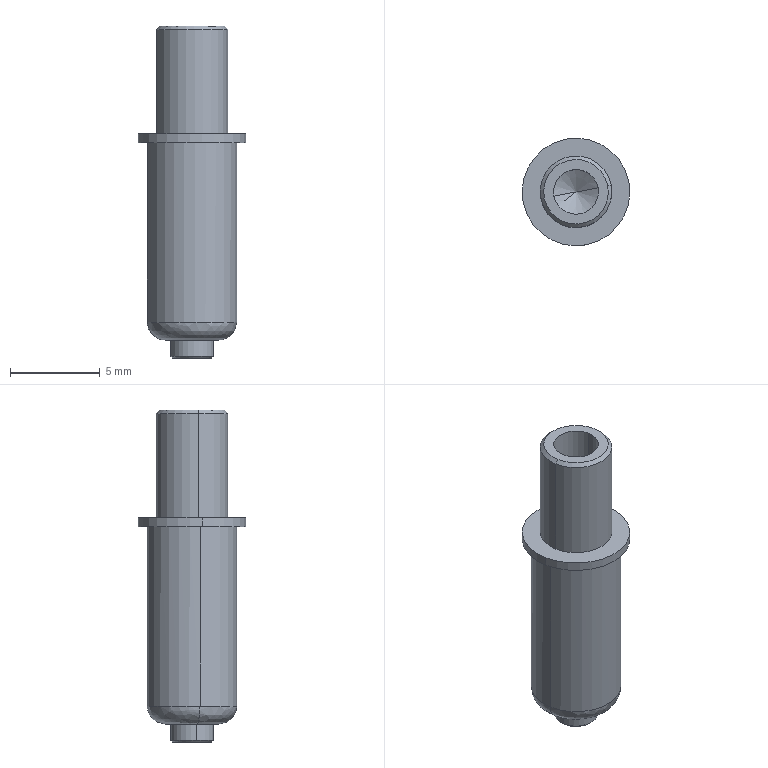Component | SolidWorks | F01AE00111-A2000-21TopEdgeAssembly-1_F01AE00111-A2000-19TopEdgeRollerAssembly-1_ElasticPIN5N--1 | 1 solid | 23 faces | box 6 x 6 x 18.5 mm | volume 274 mm3 | cylinder 10 | cone 6 | plane 5 | spline 2 | commonest cylinder face diameters 2.5 x2 4 x2 5 x2 6 x2 2.4 x2
STEP:
#1=CARTESIAN_POINT('',(-5.052,3.469,-15.668));
#2=VERTEX_POINT('',#1);
#3=CARTESIAN_POINT('',(-4.936,3.491,-15.668));
#4=VERTEX_POINT('',#3);
#5=CARTESIAN_POINT('',(-5.052,3.469,-15.668));
#6=CARTESIAN_POINT('',(-5.03,3.355,-15.668));
#7=CARTESIAN_POINT('',(-4.916,3.376,-15.668));
#8=CARTESIAN_POINT('',(-4.936,3.491,-15.668));
#9=(BOUNDED_CURVE()B_SPLINE_CURVE(3,(#5,#6,#7,#8),.UNSPECIFIED.,.F.,.T.)B_SPLINE_CURVE_WITH_KNOTS((4,4),(0.,0.9952),.UNSPECIFIED.)CURVE()GEOMETRIC_REPRESENTATION_ITEM()RATIONAL_B_SPLINE_CURVE((1.,0.3384,0.3384,1.))REPRESENTATION_ITEM(''));
#10=EDGE_CURVE('',#2,#4,#9,.T.);
#11=ORIENTED_EDGE('',*,*,#10,.T.);
#12=CARTESIAN_POINT('',(-4.897,3.498,-15.629));
#13=VERTEX_POINT('',#12);
#14=CARTESIAN_POINT('',(-4.936,3.491,-15.629));
#15=DIRECTION('',(0.1761,-0.9844,-0.));
#16=DIRECTION('',(0.9844,0.1761,0.));
#17=AXIS2_PLACEMENT_3D('',#14,#15,#16);
#18=CIRCLE('',#17,0.03937);
#19=EDGE_CURVE('',#4,#13,#18,.T.);
#20=ORIENTED_EDGE('',*,*,#19,.T.);
#21=CARTESIAN_POINT('',(-5.091,3.462,-15.629));
#22=VERTEX_POINT('',#21);
#23=CARTESIAN_POINT('',(-4.994,3.481,-15.629));
#24=DIRECTION('',(-0.,-0.,1.));
#25=DIRECTION('',(-0.9816,-0.1909,0.));
#26=AXIS2_PLACEMENT_3D('',#23,#24,#25);
#27=CIRCLE('',#26,0.09843);
#28=EDGE_CURVE('',#22,#13,#27,.T.);
#29=ORIENTED_EDGE('',*,*,#28,.F.);
#30=CARTESIAN_POINT('',(-5.091,3.463,-15.629));
#31=VERTEX_POINT('',#30);
#32=CARTESIAN_POINT('',(-4.994,3.481,-15.629));
#33=DIRECTION('',(-0.,-0.,1.));
#34=DIRECTION('',(-0.9816,-0.1909,0.));
#35=AXIS2_PLACEMENT_3D('',#32,#33,#34);
#36=CIRCLE('',#35,0.09843);
#37=EDGE_CURVE('',#31,#22,#36,.T.);
#38=ORIENTED_EDGE('',*,*,#37,.F.);
#39=CARTESIAN_POINT('',(-5.052,3.47,-15.668));
#40=VERTEX_POINT('',#39);
#41=CARTESIAN_POINT('',(-5.052,3.47,-15.629));
#42=DIRECTION('',(-0.1761,0.9844,0.));
#43=DIRECTION('',(-0.9844,-0.1761,0.));
#44=AXIS2_PLACEMENT_3D('',#41,#42,#43);
#45=CIRCLE('',#44,0.03937);
#46=EDGE_CURVE('',#40,#31,#45,.T.);
#47=ORIENTED_EDGE('',*,*,#46,.F.);
#48=CARTESIAN_POINT('',(-5.052,3.469,-15.668));
#49=CARTESIAN_POINT('',(-5.052,3.47,-15.668));
#50=CARTESIAN_POINT('',(-5.052,3.47,-15.668));
#51=CARTESIAN_POINT('',(-5.052,3.47,-15.668));
#52=B_SPLINE_CURVE_WITH_KNOTS('',3,(#48,#49,#50,#51),.UNSPECIFIED.,.F.,.F.,(4,4),(0.,0.004937),.UNSPECIFIED.);
#53=EDGE_CURVE('',#2,#40,#52,.T.);
#54=ORIENTED_EDGE('',*,*,#53,.F.);
#55=EDGE_LOOP('',(#11,#20,#29,#38,#47,#54));
#56=FACE_OUTER_BOUND('',#55,.T.);
#57=CARTESIAN_POINT('',(-4.936,3.491,-15.668));
#58=CARTESIAN_POINT('',(-4.93,3.457,-15.668));
#59=CARTESIAN_POINT('',(-4.95,3.429,-15.668));
#60=CARTESIAN_POINT('',(-4.984,3.423,-15.668));
#61=CARTESIAN_POINT('',(-5.018,3.417,-15.668));
#62=CARTESIAN_POINT('',(-5.046,3.436,-15.668));
#63=CARTESIAN_POINT('',(-5.052,3.47,-15.668));
#64=CARTESIAN_POINT('',(-4.914,3.495,-15.669));
#65=CARTESIAN_POINT('',(-4.905,3.448,-15.669));
#66=CARTESIAN_POINT('',(-4.933,3.408,-15.669));
#67=CARTESIAN_POINT('',(-4.98,3.4,-15.669));
#68=CARTESIAN_POINT('',(-5.027,3.392,-15.669));
#69=CARTESIAN_POINT('',(-5.066,3.419,-15.669));
#70=CARTESIAN_POINT('',(-5.075,3.466,-15.669));
#71=CARTESIAN_POINT('',(-4.897,3.498,-15.652));
#72=CARTESIAN_POINT('',(-4.887,3.441,-15.652));
#73=CARTESIAN_POINT('',(-4.92,3.394,-15.652));
#74=CARTESIAN_POINT('',(-4.977,3.384,-15.652));
#75=CARTESIAN_POINT('',(-5.034,3.374,-15.652));
#76=CARTESIAN_POINT('',(-5.081,3.407,-15.652));
#77=CARTESIAN_POINT('',(-5.091,3.463,-15.652));
#78=CARTESIAN_POINT('',(-4.897,3.498,-15.629));
#79=CARTESIAN_POINT('',(-4.887,3.441,-15.629));
#80=CARTESIAN_POINT('',(-4.92,3.394,-15.629));
#81=CARTESIAN_POINT('',(-4.977,3.384,-15.629));
#82=CARTESIAN_POINT('',(-5.034,3.374,-15.629));
#83=CARTESIAN_POINT('',(-5.081,3.407,-15.629));
#84=CARTESIAN_POINT('',(-5.091,3.463,-15.629));
#85=(BOUNDED_SURFACE()B_SPLINE_SURFACE(3,3,((#57,#58,#59,#60,#61,#62,#63),(#64,#65,#66,#67,#68,#69,#70),(#71,#72,#73,#74,#75,#76,#77),(#78,#79,#80,#81,#82,#83,#84)),.UNSPECIFIED.,.F.,.F.,.T.)B_SPLINE_SURFACE_WITH_KNOTS((4,4),(4,3,4),(0.,1.),(0.,0.5,1.),.UNSPECIFIED.)GEOMETRIC_REPRESENTATION_ITEM()RATIONAL_B_SPLINE_SURFACE(((1.,0.8047,0.8047,1.,0.8047,0.8047,1.),(0.8025,0.6458,0.6458,0.8025,0.6458,0.6458,0.8025),(0.8025,0.6458,0.6458,0.8025,0.6458,0.6458,0.8025),(1.,0.8047,0.8047,1.,0.8047,0.8047,1.)))REPRESENTATION_ITEM('')SURFACE());
#86=ADVANCED_FACE('',(#56),#85,.T.);
#87=CARTESIAN_POINT('',(-4.925,3.494,-14.979));
#88=VERTEX_POINT('',#87);
#89=CARTESIAN_POINT('',(-5.064,3.467,-14.979));
#90=VERTEX_POINT('',#89);
#91=CARTESIAN_POINT('',(-4.994,3.481,-14.979));
#92=DIRECTION('',(-0.,-0.,1.));
#93=DIRECTION('',(0.9816,0.1909,0.));
#94=AXIS2_PLACEMENT_3D('',#91,#92,#93);
#95=CIRCLE('',#94,0.07087);
#96=EDGE_CURVE('',#88,#90,#95,.T.);
#97=ORIENTED_EDGE('',*,*,#96,.F.);
#98=CARTESIAN_POINT('',(-4.917,3.496,-14.987));
#99=VERTEX_POINT('',#98);
#100=CARTESIAN_POINT('',(-4.925,3.494,-14.979));
#101=DIRECTION('',(0.6941,0.135,-0.7071));
#102=VECTOR('',#101,39.37);
#103=LINE('',#100,#102);
#104=EDGE_CURVE('',#88,#99,#103,.T.);
#105=ORIENTED_EDGE('',*,*,#104,.T.);
#106=CARTESIAN_POINT('',(-5.071,3.466,-14.987));
#107=VERTEX_POINT('',#106);
#108=CARTESIAN_POINT('',(-4.994,3.481,-14.987));
#109=DIRECTION('',(0.,0.,-1.));
#110=DIRECTION('',(0.9816,0.1909,0.));
#111=AXIS2_PLACEMENT_3D('',#108,#109,#110);
#112=CIRCLE('',#111,0.07874);
#113=EDGE_CURVE('',#107,#99,#112,.T.);
#114=ORIENTED_EDGE('',*,*,#113,.F.);
#115=CARTESIAN_POINT('',(-5.064,3.467,-14.979));
#116=DIRECTION('',(-0.6941,-0.135,-0.7071));
#117=VECTOR('',#116,39.37);
#118=LINE('',#115,#117);
#119=EDGE_CURVE('',#90,#107,#118,.T.);
#120=ORIENTED_EDGE('',*,*,#119,.F.);
#121=EDGE_LOOP('',(#97,#105,#114,#120));
#122=FACE_OUTER_BOUND('',#121,.T.);
#123=CARTESIAN_POINT('',(-4.994,3.481,-14.979));
#124=DIRECTION('',(0.,0.,-1.));
#125=DIRECTION('',(-0.9816,-0.1909,0.));
#126=AXIS2_PLACEMENT_3D('',#123,#124,#125);
#127=CONICAL_SURFACE('',#126,0.07087,0.7854);
#128=ADVANCED_FACE('',(#122),#127,.T.);
#129=CARTESIAN_POINT('',(-5.042,3.471,-15.235));
#130=VERTEX_POINT('',#129);
#131=CARTESIAN_POINT('',(-4.946,3.49,-15.235));
#132=VERTEX_POINT('',#131);
#133=CARTESIAN_POINT('',(-4.994,3.481,-15.235));
#134=DIRECTION('',(-0.,-0.,1.));
#135=DIRECTION('',(0.9816,0.1909,0.));
#136=AXIS2_PLACEMENT_3D('',#133,#134,#135);
#137=CIRCLE('',#136,0.04921);
#138=EDGE_CURVE('',#130,#132,#137,.T.);
#139=ORIENTED_EDGE('',*,*,#138,.F.);
#140=CARTESIAN_POINT('',(-5.042,3.471,-14.979));
#141=VERTEX_POINT('',#140);
#142=CARTESIAN_POINT('',(-5.042,3.471,-14.979));
#143=DIRECTION('',(-0.,-0.,1.));
#144=VECTOR('',#143,39.37);
#145=LINE('',#142,#144);
#146=EDGE_CURVE('',#130,#141,#145,.T.);
#147=ORIENTED_EDGE('',*,*,#146,.T.);
#148=CARTESIAN_POINT('',(-4.946,3.49,-14.979));
#149=VERTEX_POINT('',#148);
#150=CARTESIAN_POINT('',(-4.994,3.481,-14.979));
#151=DIRECTION('',(-0.,-0.,1.));
#152=DIRECTION('',(0.9816,0.1909,0.));
#153=AXIS2_PLACEMENT_3D('',#150,#151,#152);
#154=CIRCLE('',#153,0.04921);
#155=EDGE_CURVE('',#141,#149,#154,.T.);
#156=ORIENTED_EDGE('',*,*,#155,.T.);
#157=CARTESIAN_POINT('',(-4.946,3.49,-14.979));
#158=DIRECTION('',(-0.,-0.,1.));
#159=VECTOR('',#158,39.37);
#160=LINE('',#157,#159);
#161=EDGE_CURVE('',#132,#149,#160,.T.);
#162=ORIENTED_EDGE('',*,*,#161,.F.);
#163=EDGE_LOOP('',(#139,#147,#156,#162));
#164=FACE_OUTER_BOUND('',#163,.T.);
#165=CARTESIAN_POINT('',(-4.994,3.481,-14.979));
#166=DIRECTION('',(-0.,-0.,1.));
#167=DIRECTION('',(0.9816,0.1909,0.));
#168=AXIS2_PLACEMENT_3D('',#165,#166,#167);
#169=CYLINDRICAL_SURFACE('',#168,0.04921);
#170=ADVANCED_FACE('',(#164),#169,.F.);
#171=CARTESIAN_POINT('',(-4.994,3.481,-15.265));
#172=VERTEX_POINT('',#171);
#173=CARTESIAN_POINT('',(-4.946,3.49,-15.235));
#174=DIRECTION('',(0.8414,0.1637,0.515));
#175=VECTOR('',#174,39.37);
#176=LINE('',#173,#175);
#177=EDGE_CURVE('',#172,#132,#176,.T.);
#178=ORIENTED_EDGE('',*,*,#177,.F.);
#179=CARTESIAN_POINT('',(-5.042,3.471,-15.235));
#180=DIRECTION('',(-0.8414,-0.1637,0.515));
#181=VECTOR('',#180,39.37);
#182=LINE('',#179,#181);
#183=EDGE_CURVE('',#172,#130,#182,.T.);
#184=ORIENTED_EDGE('',*,*,#183,.T.);
#185=ORIENTED_EDGE('',*,*,#138,.T.);
#186=EDGE_LOOP('',(#178,#184,#185));
#187=FACE_OUTER_BOUND('',#186,.T.);
#188=CARTESIAN_POINT('',(-4.994,3.481,-15.235));
#189=DIRECTION('',(-0.,-0.,1.));
#190=DIRECTION('',(0.9816,0.1909,0.));
#191=AXIS2_PLACEMENT_3D('',#188,#189,#190);
#192=CONICAL_SURFACE('',#191,0.04921,1.03);
#193=ADVANCED_FACE('',(#187),#192,.F.);
#194=ORIENTED_EDGE('',*,*,#113,.T.);
#195=CARTESIAN_POINT('',(-4.917,3.496,-15.216));
#196=VERTEX_POINT('',#195);
#197=CARTESIAN_POINT('',(-4.917,3.496,-14.979));
#198=DIRECTION('',(0.,0.,-1.));
#199=VECTOR('',#198,39.37);
#200=LINE('',#197,#199);
#201=EDGE_CURVE('',#99,#196,#200,.T.);
#202=ORIENTED_EDGE('',*,*,#201,.T.);
#203=CARTESIAN_POINT('',(-5.071,3.466,-15.216));
#204=VERTEX_POINT('',#203);
#205=CARTESIAN_POINT('',(-4.994,3.481,-15.216));
#206=DIRECTION('',(-0.,-0.,1.));
#207=DIRECTION('',(-0.9816,-0.1909,0.));
#208=AXIS2_PLACEMENT_3D('',#205,#206,#207);
#209=CIRCLE('',#208,0.07874);
#210=EDGE_CURVE('',#196,#204,#209,.T.);
#211=ORIENTED_EDGE('',*,*,#210,.T.);
#212=CARTESIAN_POINT('',(-5.071,3.466,-14.979));
#213=DIRECTION('',(0.,0.,-1.));
#214=VECTOR('',#213,39.37);
#215=LINE('',#212,#214);
#216=EDGE_CURVE('',#107,#204,#215,.T.);
#217=ORIENTED_EDGE('',*,*,#216,.F.);
#218=EDGE_LOOP('',(#194,#202,#211,#217));
#219=FACE_OUTER_BOUND('',#218,.T.);
#220=CARTESIAN_POINT('',(-4.994,3.481,-14.979));
#221=DIRECTION('',(0.,0.,-1.));
#222=DIRECTION('',(-0.9816,-0.1909,0.));
#223=AXIS2_PLACEMENT_3D('',#220,#221,#222);
#224=CYLINDRICAL_SURFACE('',#223,0.07874);
#225=ADVANCED_FACE('',(#219),#224,.T.);
#226=CARTESIAN_POINT('',(-5.091,3.462,-15.235));
#227=VERTEX_POINT('',#226);
#228=CARTESIAN_POINT('',(-4.898,3.499,-15.235));
#229=VERTEX_POINT('',#228);
#230=CARTESIAN_POINT('',(-4.994,3.481,-15.235));
#231=DIRECTION('',(0.,0.,-1.));
#232=DIRECTION('',(-0.9816,-0.1909,0.));
#233=AXIS2_PLACEMENT_3D('',#230,#231,#232);
#234=CIRCLE('',#233,0.09843);
#235=EDGE_CURVE('',#227,#229,#234,.T.);
#236=ORIENTED_EDGE('',*,*,#235,.T.);
#237=CARTESIAN_POINT('',(-4.898,3.499,-15.629));
#238=VERTEX_POINT('',#237);
#239=CARTESIAN_POINT('',(-4.898,3.499,-14.777));
#240=DIRECTION('',(0.,0.,-1.));
#241=VECTOR('',#240,39.37);
#242=LINE('',#239,#241);
#243=EDGE_CURVE('',#229,#238,#242,.T.);
#244=ORIENTED_EDGE('',*,*,#243,.T.);
#245=CARTESIAN_POINT('',(-4.994,3.481,-15.629));
#246=DIRECTION('',(-0.,-0.,1.));
#247=DIRECTION('',(-0.9816,-0.1909,0.));
#248=AXIS2_PLACEMENT_3D('',#245,#246,#247);
#249=CIRCLE('',#248,0.09843);
#250=EDGE_CURVE('',#238,#31,#249,.T.);
#251=ORIENTED_EDGE('',*,*,#250,.T.);
#252=ORIENTED_EDGE('',*,*,#37,.T.);
#253=CARTESIAN_POINT('',(-5.091,3.462,-14.777));
#254=DIRECTION('',(0.,0.,-1.));
#255=VECTOR('',#254,39.37);
#256=LINE('',#253,#255);
#257=EDGE_CURVE('',#227,#22,#256,.T.);
#258=ORIENTED_EDGE('',*,*,#257,.F.);
#259=EDGE_LOOP('',(#236,#244,#251,#252,#258));
#260=FACE_OUTER_BOUND('',#259,.T.);
#261=CARTESIAN_POINT('',(-4.994,3.481,-14.777));
#262=DIRECTION('',(0.,0.,-1.));
#263=DIRECTION('',(-0.9816,-0.1909,0.));
#264=AXIS2_PLACEMENT_3D('',#261,#262,#263);
#265=CYLINDRICAL_SURFACE('',#264,0.09843);
#266=ADVANCED_FACE('',(#260),#265,.T.);
#267=CARTESIAN_POINT('',(-5.11,3.458,-15.216));
#268=VERTEX_POINT('',#267);
#269=CARTESIAN_POINT('',(-4.878,3.503,-15.216));
#270=VERTEX_POINT('',#269);
#271=CARTESIAN_POINT('',(-4.994,3.481,-15.216));
#272=DIRECTION('',(0.,0.,-1.));
#273=DIRECTION('',(-0.9816,-0.1909,0.));
#274=AXIS2_PLACEMENT_3D('',#271,#272,#273);
#275=CIRCLE('',#274,0.1181);
#276=EDGE_CURVE('',#268,#270,#275,.T.);
#277=ORIENTED_EDGE('',*,*,#276,.T.);
#278=CARTESIAN_POINT('',(-4.878,3.503,-15.235));
#279=VERTEX_POINT('',#278);
#280=CARTESIAN_POINT('',(-4.878,3.503,-14.777));
#281=DIRECTION('',(0.,0.,-1.));
#282=VECTOR('',#281,39.37);
#283=LINE('',#280,#282);
#284=EDGE_CURVE('',#270,#279,#283,.T.);
#285=ORIENTED_EDGE('',*,*,#284,.T.);
#286=CARTESIAN_POINT('',(-5.11,3.458,-15.235));
#287=VERTEX_POINT('',#286);
#288=CARTESIAN_POINT('',(-4.994,3.481,-15.235));
#289=DIRECTION('',(0.,0.,-1.));
#290=DIRECTION('',(-0.9816,-0.1909,0.));
#291=AXIS2_PLACEMENT_3D('',#288,#289,#290);
#292=CIRCLE('',#291,0.1181);
#293=EDGE_CURVE('',#287,#279,#292,.T.);
#294=ORIENTED_EDGE('',*,*,#293,.F.);
#295=CARTESIAN_POINT('',(-5.11,3.458,-14.777));
#296=DIRECTION('',(0.,0.,-1.));
#297=VECTOR('',#296,39.37);
#298=LINE('',#295,#297);
#299=EDGE_CURVE('',#268,#287,#298,.T.);
#300=ORIENTED_EDGE('',*,*,#299,.F.);
#301=EDGE_LOOP('',(#277,#285,#294,#300));
#302=FACE_OUTER_BOUND('',#301,.T.);
#303=CARTESIAN_POINT('',(-4.994,3.481,-14.777));
#304=DIRECTION('',(0.,0.,-1.));
#305=DIRECTION('',(-0.9816,-0.1909,0.));
#306=AXIS2_PLACEMENT_3D('',#303,#304,#305);
#307=CYLINDRICAL_SURFACE('',#306,0.1181);
#308=ADVANCED_FACE('',(#302),#307,.T.);
#309=CARTESIAN_POINT('',(-4.948,3.49,-15.668));
#310=VERTEX_POINT('',#309);
#311=CARTESIAN_POINT('',(-5.041,3.472,-15.668));
#312=VERTEX_POINT('',#311);
#313=CARTESIAN_POINT('',(-4.994,3.481,-15.668));
#314=DIRECTION('',(-0.,-0.,1.));
#315=DIRECTION('',(-0.9816,-0.1909,0.));
#316=AXIS2_PLACEMENT_3D('',#313,#314,#315);
#317=CIRCLE('',#316,0.04724);
#318=EDGE_CURVE('',#310,#312,#317,.T.);
#319=ORIENTED_EDGE('',*,*,#318,.F.);
#320=CARTESIAN_POINT('',(-4.948,3.49,-15.704));
#321=VERTEX_POINT('',#320);
#322=CARTESIAN_POINT('',(-4.948,3.49,-14.777));
#323=DIRECTION('',(0.,0.,-1.));
#324=VECTOR('',#323,39.37);
#325=LINE('',#322,#324);
#326=EDGE_CURVE('',#310,#321,#325,.T.);
#327=ORIENTED_EDGE('',*,*,#326,.T.);
#328=CARTESIAN_POINT('',(-5.041,3.472,-15.704));
#329=VERTEX_POINT('',#328);
#330=CARTESIAN_POINT('',(-4.994,3.481,-15.704));
#331=DIRECTION('',(-0.,-0.,1.));
#332=DIRECTION('',(-0.9816,-0.1909,0.));
#333=AXIS2_PLACEMENT_3D('',#330,#331,#332);
#334=CIRCLE('',#333,0.04724);
#335=EDGE_CURVE('',#321,#329,#334,.T.);
#336=ORIENTED_EDGE('',*,*,#335,.T.);
#337=CARTESIAN_POINT('',(-5.041,3.472,-14.777));
#338=DIRECTION('',(0.,0.,-1.));
#339=VECTOR('',#338,39.37);
#340=LINE('',#337,#339);
#341=EDGE_CURVE('',#312,#329,#340,.T.);
#342=ORIENTED_EDGE('',*,*,#341,.F.);
#343=EDGE_LOOP('',(#319,#327,#336,#342));
#344=FACE_OUTER_BOUND('',#343,.T.);
#345=CARTESIAN_POINT('',(-4.994,3.481,-14.777));
#346=DIRECTION('',(0.,0.,-1.));
#347=DIRECTION('',(-0.9816,-0.1909,0.));
#348=AXIS2_PLACEMENT_3D('',#345,#346,#347);
#349=CYLINDRICAL_SURFACE('',#348,0.04724);
#350=ADVANCED_FACE('',(#344),#349,.T.);
#351=CARTESIAN_POINT('',(-4.952,3.489,-15.708));
#352=VERTEX_POINT('',#351);
#353=CARTESIAN_POINT('',(-5.037,3.472,-15.708));
#354=VERTEX_POINT('',#353);
#355=CARTESIAN_POINT('',(-4.994,3.481,-15.708));
#356=DIRECTION('',(-0.,-0.,1.));
#357=DIRECTION('',(0.9816,0.1909,0.));
#358=AXIS2_PLACEMENT_3D('',#355,#356,#357);
#359=CIRCLE('',#358,0.04331);
#360=EDGE_CURVE('',#352,#354,#359,.T.);
#361=ORIENTED_EDGE('',*,*,#360,.T.);
#362=CARTESIAN_POINT('',(-5.041,3.472,-15.704));
#363=DIRECTION('',(-0.6941,-0.135,0.7071));
#364=VECTOR('',#363,39.37);
#365=LINE('',#362,#364);
#366=EDGE_CURVE('',#354,#329,#365,.T.);
#367=ORIENTED_EDGE('',*,*,#366,.T.);
#368=ORIENTED_EDGE('',*,*,#335,.F.);
#369=CARTESIAN_POINT('',(-4.948,3.49,-15.704));
#370=DIRECTION('',(0.6941,0.135,0.7071));
#371=VECTOR('',#370,39.37);
#372=LINE('',#369,#371);
#373=EDGE_CURVE('',#352,#321,#372,.T.);
#374=ORIENTED_EDGE('',*,*,#373,.F.);
#375=EDGE_LOOP('',(#361,#367,#368,#374));
#376=FACE_OUTER_BOUND('',#375,.T.);
#377=CARTESIAN_POINT('',(-4.994,3.481,-15.704));
#378=DIRECTION('',(-0.,-0.,1.));
#379=DIRECTION('',(0.9816,0.1909,0.));
#380=AXIS2_PLACEMENT_3D('',#377,#378,#379);
#381=CONICAL_SURFACE('',#380,0.04724,0.7854);
#382=ADVANCED_FACE('',(#376),#381,.T.);
#383=ORIENTED_EDGE('',*,*,#276,.F.);
#384=CARTESIAN_POINT('',(-4.994,3.481,-15.216));
#385=DIRECTION('',(0.,0.,-1.));
#386=DIRECTION('',(-0.9816,-0.1909,0.));
#387=AXIS2_PLACEMENT_3D('',#384,#385,#386);
#388=CIRCLE('',#387,0.1181);
#389=EDGE_CURVE('',#270,#268,#388,.T.);
#390=ORIENTED_EDGE('',*,*,#389,.F.);
#391=EDGE_LOOP('',(#383,#390));
#392=FACE_OUTER_BOUND('',#391,.T.);
#393=CARTESIAN_POINT('',(-4.994,3.481,-15.216));
#394=DIRECTION('',(-0.,-0.,1.));
#395=DIRECTION('',(-0.9816,-0.1909,0.));
#396=AXIS2_PLACEMENT_3D('',#393,#394,#395);
#397=CIRCLE('',#396,0.07874);
#398=EDGE_CURVE('',#204,#196,#397,.T.);
#399=ORIENTED_EDGE('',*,*,#398,.F.);
#400=ORIENTED_EDGE('',*,*,#210,.F.);
#401=EDGE_LOOP('',(#399,#400));
#402=FACE_BOUND('',#401,.T.);
#403=CARTESIAN_POINT('',(-4.994,3.481,-15.216));
#404=DIRECTION('',(0.,0.,-1.));
#405=DIRECTION('',(-0.9816,-0.1909,-0.));
#406=AXIS2_PLACEMENT_3D('',#403,#404,#405);
#407=PLANE('',#406);
#408=ADVANCED_FACE('',(#392,#402),#407,.F.);
#409=ORIENTED_EDGE('',*,*,#243,.F.);
#410=CARTESIAN_POINT('',(-4.994,3.481,-15.235));
#411=DIRECTION('',(0.,0.,-1.));
#412=DIRECTION('',(-0.9816,-0.1909,0.));
#413=AXIS2_PLACEMENT_3D('',#410,#411,#412);
#414=CIRCLE('',#413,0.09843);
#415=EDGE_CURVE('',#229,#227,#414,.T.);
#416=ORIENTED_EDGE('',*,*,#415,.T.);
#417=ORIENTED_EDGE('',*,*,#257,.T.);
#418=ORIENTED_EDGE('',*,*,#28,.T.);
#419=CARTESIAN_POINT('',(-4.994,3.481,-15.629));
#420=DIRECTION('',(-0.,-0.,1.));
#421=DIRECTION('',(-0.9816,-0.1909,0.));
#422=AXIS2_PLACEMENT_3D('',#419,#420,#421);
#423=CIRCLE('',#422,0.09843);
#424=EDGE_CURVE('',#13,#238,#423,.T.);
#425=ORIENTED_EDGE('',*,*,#424,.T.);
#426=EDGE_LOOP('',(#409,#416,#417,#418,#425));
#427=FACE_OUTER_BOUND('',#426,.T.);
#428=CARTESIAN_POINT('',(-4.994,3.481,-14.777));
#429=DIRECTION('',(0.,0.,-1.));
#430=DIRECTION('',(-0.9816,-0.1909,0.));
#431=AXIS2_PLACEMENT_3D('',#428,#429,#430);
#432=CYLINDRICAL_SURFACE('',#431,0.09843);
#433=ADVANCED_FACE('',(#427),#432,.T.);
#434=ORIENTED_EDGE('',*,*,#19,.F.);
#435=CARTESIAN_POINT('',(-4.936,3.492,-15.668));
#436=VERTEX_POINT('',#435);
#437=CARTESIAN_POINT('',(-4.936,3.491,-15.668));
#438=CARTESIAN_POINT('',(-4.936,3.491,-15.668));
#439=CARTESIAN_POINT('',(-4.936,3.492,-15.668));
#440=CARTESIAN_POINT('',(-4.936,3.492,-15.668));
#441=(BOUNDED_CURVE()B_SPLINE_CURVE(3,(#437,#438,#439,#440),.UNSPECIFIED.,.F.,.T.)B_SPLINE_CURVE_WITH_KNOTS((4,4),(0.9952,1.),.UNSPECIFIED.)CURVE()GEOMETRIC_REPRESENTATION_ITEM()RATIONAL_B_SPLINE_CURVE((1.,1.,1.,1.))REPRESENTATION_ITEM(''));
#442=EDGE_CURVE('',#4,#436,#441,.T.);
#443=ORIENTED_EDGE('',*,*,#442,.T.);
#444=CARTESIAN_POINT('',(-5.052,3.47,-15.668));
#445=CARTESIAN_POINT('',(-5.053,3.474,-15.668));
#446=CARTESIAN_POINT('',(-5.053,3.479,-15.668));
#447=CARTESIAN_POINT('',(-5.053,3.485,-15.668));
#448=CARTESIAN_POINT('',(-5.053,3.489,-15.668));
#449=CARTESIAN_POINT('',(-5.052,3.49,-15.668));
#450=CARTESIAN_POINT('',(-5.05,3.5,-15.668));
#451=CARTESIAN_POINT('',(-5.047,3.508,-15.668));
#452=CARTESIAN_POINT('',(-5.04,3.518,-15.668));
#453=CARTESIAN_POINT('',(-5.037,3.522,-15.668));
#454=CARTESIAN_POINT('',(-5.031,3.527,-15.668));
#455=CARTESIAN_POINT('',(-5.029,3.528,-15.668));
#456=CARTESIAN_POINT('',(-5.027,3.53,-15.668));
#457=CARTESIAN_POINT('',(-5.026,3.53,-15.668));
#458=CARTESIAN_POINT('',(-5.019,3.535,-15.668));
#459=CARTESIAN_POINT('',(-5.012,3.537,-15.668));
#460=CARTESIAN_POINT('',(-5.001,3.539,-15.668));
#461=CARTESIAN_POINT('',(-4.996,3.54,-15.668));
#462=CARTESIAN_POINT('',(-4.989,3.54,-15.668));
#463=CARTESIAN_POINT('',(-4.987,3.539,-15.668));
#464=CARTESIAN_POINT('',(-4.985,3.539,-15.668));
#465=CARTESIAN_POINT('',(-4.984,3.539,-15.668));
#466=CARTESIAN_POINT('',(-4.975,3.537,-15.668));
#467=CARTESIAN_POINT('',(-4.968,3.534,-15.668));
#468=CARTESIAN_POINT('',(-4.958,3.527,-15.668));
#469=CARTESIAN_POINT('',(-4.953,3.523,-15.668));
#470=CARTESIAN_POINT('',(-4.948,3.518,-15.668));
#471=CARTESIAN_POINT('',(-4.947,3.516,-15.668));
#472=CARTESIAN_POINT('',(-4.945,3.514,-15.668));
#473=CARTESIAN_POINT('',(-4.945,3.513,-15.668));
#474=CARTESIAN_POINT('',(-4.94,3.506,-15.668));
#475=CARTESIAN_POINT('',(-4.938,3.499,-15.668));
#476=CARTESIAN_POINT('',(-4.936,3.492,-15.668));
#477=B_SPLINE_CURVE_WITH_KNOTS('',3,(#444,#445,#446,#447,#448,#449,#450,#451,#452,#453,#454,#455,#456,#457,#458,#459,#460,#461,#462,#463,#464,#465,#466,#467,#468,#469,#470,#471,#472,#473,#474,#475,#476),.UNSPECIFIED.,.F.,.F.,(4,1,2,2,2,1,1,2,2,2,1,1,2,2,2,1,1,2,2,4),(0.004937,0.06713,0.09822,0.1293,0.2537,0.3159,0.347,0.3625,0.3781,0.5025,0.5647,0.5958,0.6113,0.6269,0.7512,0.8134,0.8445,0.8601,0.8756,1.),.UNSPECIFIED.);
#478=EDGE_CURVE('',#40,#436,#477,.T.);
#479=ORIENTED_EDGE('',*,*,#478,.F.);
#480=ORIENTED_EDGE('',*,*,#46,.T.);
#481=ORIENTED_EDGE('',*,*,#250,.F.);
#482=ORIENTED_EDGE('',*,*,#424,.F.);
#483=EDGE_LOOP('',(#434,#443,#479,#480,#481,#482));
#484=FACE_OUTER_BOUND('',#483,.T.);
#485=CARTESIAN_POINT('',(-5.052,3.469,-15.668));
#486=CARTESIAN_POINT('',(-5.058,3.503,-15.668));
#487=CARTESIAN_POINT('',(-5.039,3.532,-15.668));
#488=CARTESIAN_POINT('',(-5.005,3.538,-15.668));
#489=CARTESIAN_POINT('',(-4.971,3.545,-15.668));
#490=CARTESIAN_POINT('',(-4.943,3.525,-15.668));
#491=CARTESIAN_POINT('',(-4.936,3.491,-15.668));
#492=CARTESIAN_POINT('',(-5.075,3.465,-15.669));
#493=CARTESIAN_POINT('',(-5.084,3.512,-15.669));
#494=CARTESIAN_POINT('',(-5.057,3.552,-15.669));
#495=CARTESIAN_POINT('',(-5.009,3.561,-15.669));
#496=CARTESIAN_POINT('',(-4.962,3.57,-15.669));
#497=CARTESIAN_POINT('',(-4.922,3.543,-15.669));
#498=CARTESIAN_POINT('',(-4.914,3.495,-15.669));
#499=CARTESIAN_POINT('',(-5.091,3.461,-15.652));
#500=CARTESIAN_POINT('',(-5.102,3.518,-15.652));
#501=CARTESIAN_POINT('',(-5.069,3.567,-15.652));
#502=CARTESIAN_POINT('',(-5.012,3.577,-15.652));
#503=CARTESIAN_POINT('',(-4.955,3.588,-15.652));
#504=CARTESIAN_POINT('',(-4.908,3.555,-15.652));
#505=CARTESIAN_POINT('',(-4.897,3.498,-15.652));
#506=CARTESIAN_POINT('',(-5.091,3.461,-15.629));
#507=CARTESIAN_POINT('',(-5.102,3.518,-15.629));
#508=CARTESIAN_POINT('',(-5.069,3.567,-15.629));
#509=CARTESIAN_POINT('',(-5.012,3.577,-15.629));
#510=CARTESIAN_POINT('',(-4.955,3.588,-15.629));
#511=CARTESIAN_POINT('',(-4.908,3.555,-15.629));
#512=CARTESIAN_POINT('',(-4.897,3.498,-15.629));
#513=(BOUNDED_SURFACE()B_SPLINE_SURFACE(3,3,((#485,#486,#487,#488,#489,#490,#491),(#492,#493,#494,#495,#496,#497,#498),(#499,#500,#501,#502,#503,#504,#505),(#506,#507,#508,#509,#510,#511,#512)),.UNSPECIFIED.,.F.,.F.,.T.)B_SPLINE_SURFACE_WITH_KNOTS((4,4),(4,3,4),(0.,1.),(0.,0.5,1.),.UNSPECIFIED.)GEOMETRIC_REPRESENTATION_ITEM()RATIONAL_B_SPLINE_SURFACE(((1.,0.8025,0.8025,1.,0.8025,0.8025,1.),(0.8024,0.644,0.644,0.8024,0.644,0.644,0.8024),(0.8024,0.644,0.644,0.8024,0.644,0.644,0.8024),(1.,0.8025,0.8025,1.,0.8025,0.8025,1.)))REPRESENTATION_ITEM('')SURFACE());
#514=ADVANCED_FACE('',(#484),#513,.T.);
#515=ORIENTED_EDGE('',*,*,#235,.F.);
#516=ORIENTED_EDGE('',*,*,#415,.F.);
#517=EDGE_LOOP('',(#515,#516));
#518=FACE_BOUND('',#517,.T.);
#519=ORIENTED_EDGE('',*,*,#293,.T.);
#520=CARTESIAN_POINT('',(-4.994,3.481,-15.235));
#521=DIRECTION('',(0.,0.,-1.));
#522=DIRECTION('',(-0.9816,-0.1909,0.));
#523=AXIS2_PLACEMENT_3D('',#520,#521,#522);
#524=CIRCLE('',#523,0.1181);
#525=EDGE_CURVE('',#279,#287,#524,.T.);
#526=ORIENTED_EDGE('',*,*,#525,.T.);
#527=EDGE_LOOP('',(#519,#526));
#528=FACE_OUTER_BOUND('',#527,.T.);
#529=CARTESIAN_POINT('',(-4.994,3.481,-15.235));
#530=DIRECTION('',(0.,0.,-1.));
#531=DIRECTION('',(-0.9816,-0.1909,-0.));
#532=AXIS2_PLACEMENT_3D('',#529,#530,#531);
#533=PLANE('',#532);
#534=ADVANCED_FACE('',(#518,#528),#533,.T.);
#535=CARTESIAN_POINT('',(-4.994,3.481,-15.668));
#536=DIRECTION('',(-0.,-0.,1.));
#537=DIRECTION('',(-0.9816,-0.1909,0.));
#538=AXIS2_PLACEMENT_3D('',#535,#536,#537);
#539=CIRCLE('',#538,0.04724);
#540=EDGE_CURVE('',#312,#310,#539,.T.);
#541=ORIENTED_EDGE('',*,*,#540,.T.);
#542=ORIENTED_EDGE('',*,*,#318,.T.);
#543=EDGE_LOOP('',(#541,#542));
#544=FACE_BOUND('',#543,.T.);
#545=ORIENTED_EDGE('',*,*,#53,.T.);
#546=ORIENTED_EDGE('',*,*,#478,.T.);
#547=ORIENTED_EDGE('',*,*,#442,.F.);
#548=ORIENTED_EDGE('',*,*,#10,.F.);
#549=EDGE_LOOP('',(#545,#546,#547,#548));
#550=FACE_OUTER_BOUND('',#549,.T.);
#551=CARTESIAN_POINT('',(-4.994,3.481,-15.668));
#552=DIRECTION('',(0.,0.,-1.));
#553=DIRECTION('',(-0.9816,-0.1909,-0.));
#554=AXIS2_PLACEMENT_3D('',#551,#552,#553);
#555=PLANE('',#554);
#556=ADVANCED_FACE('',(#544,#550),#555,.T.);
#557=ORIENTED_EDGE('',*,*,#284,.F.);
#558=ORIENTED_EDGE('',*,*,#389,.T.);
#559=ORIENTED_EDGE('',*,*,#299,.T.);
#560=ORIENTED_EDGE('',*,*,#525,.F.);
#561=EDGE_LOOP('',(#557,#558,#559,#560));
#562=FACE_OUTER_BOUND('',#561,.T.);
#563=CARTESIAN_POINT('',(-4.994,3.481,-14.777));
#564=DIRECTION('',(0.,0.,-1.));
#565=DIRECTION('',(-0.9816,-0.1909,0.));
#566=AXIS2_PLACEMENT_3D('',#563,#564,#565);
#567=CYLINDRICAL_SURFACE('',#566,0.1181);
#568=ADVANCED_FACE('',(#562),#567,.T.);
#569=ORIENTED_EDGE('',*,*,#326,.F.);
#570=ORIENTED_EDGE('',*,*,#540,.F.);
#571=ORIENTED_EDGE('',*,*,#341,.T.);
#572=CARTESIAN_POINT('',(-4.994,3.481,-15.704));
#573=DIRECTION('',(-0.,-0.,1.));
#574=DIRECTION('',(-0.9816,-0.1909,0.));
#575=AXIS2_PLACEMENT_3D('',#572,#573,#574);
#576=CIRCLE('',#575,0.04724);
#577=EDGE_CURVE('',#329,#321,#576,.T.);
#578=ORIENTED_EDGE('',*,*,#577,.T.);
#579=EDGE_LOOP('',(#569,#570,#571,#578));
#580=FACE_OUTER_BOUND('',#579,.T.);
#581=CARTESIAN_POINT('',(-4.994,3.481,-14.777));
#582=DIRECTION('',(0.,0.,-1.));
#583=DIRECTION('',(-0.9816,-0.1909,0.));
#584=AXIS2_PLACEMENT_3D('',#581,#582,#583);
#585=CYLINDRICAL_SURFACE('',#584,0.04724);
#586=ADVANCED_FACE('',(#580),#585,.T.);
#587=ORIENTED_EDGE('',*,*,#366,.F.);
#588=CARTESIAN_POINT('',(-4.994,3.481,-15.708));
#589=DIRECTION('',(-0.,-0.,1.));
#590=DIRECTION('',(0.9816,0.1909,0.));
#591=AXIS2_PLACEMENT_3D('',#588,#589,#590);
#592=CIRCLE('',#591,0.04331);
#593=EDGE_CURVE('',#354,#352,#592,.T.);
#594=ORIENTED_EDGE('',*,*,#593,.T.);
#595=ORIENTED_EDGE('',*,*,#373,.T.);
#596=ORIENTED_EDGE('',*,*,#577,.F.);
#597=EDGE_LOOP('',(#587,#594,#595,#596));
#598=FACE_OUTER_BOUND('',#597,.T.);
#599=CARTESIAN_POINT('',(-4.994,3.481,-15.704));
#600=DIRECTION('',(-0.,-0.,1.));
#601=DIRECTION('',(0.9816,0.1909,0.));
#602=AXIS2_PLACEMENT_3D('',#599,#600,#601);
#603=CONICAL_SURFACE('',#602,0.04724,0.7854);
#604=ADVANCED_FACE('',(#598),#603,.T.);
#605=ORIENTED_EDGE('',*,*,#360,.F.);
#606=ORIENTED_EDGE('',*,*,#593,.F.);
#607=EDGE_LOOP('',(#605,#606));
#608=FACE_OUTER_BOUND('',#607,.T.);
#609=CARTESIAN_POINT('',(-4.994,3.481,-15.708));
#610=DIRECTION('',(0.,0.,-1.));
#611=DIRECTION('',(-0.9816,-0.1909,-0.));
#612=AXIS2_PLACEMENT_3D('',#609,#610,#611);
#613=PLANE('',#612);
#614=ADVANCED_FACE('',(#608),#613,.T.);
#615=ORIENTED_EDGE('',*,*,#201,.F.);
#616=CARTESIAN_POINT('',(-4.994,3.481,-14.987));
#617=DIRECTION('',(0.,0.,-1.));
#618=DIRECTION('',(0.9816,0.1909,0.));
#619=AXIS2_PLACEMENT_3D('',#616,#617,#618);
#620=CIRCLE('',#619,0.07874);
#621=EDGE_CURVE('',#99,#107,#620,.T.);
#622=ORIENTED_EDGE('',*,*,#621,.T.);
#623=ORIENTED_EDGE('',*,*,#216,.T.);
#624=ORIENTED_EDGE('',*,*,#398,.T.);
#625=EDGE_LOOP('',(#615,#622,#623,#624));
#626=FACE_OUTER_BOUND('',#625,.T.);
#627=CARTESIAN_POINT('',(-4.994,3.481,-14.979));
#628=DIRECTION('',(0.,0.,-1.));
#629=DIRECTION('',(-0.9816,-0.1909,0.));
#630=AXIS2_PLACEMENT_3D('',#627,#628,#629);
#631=CYLINDRICAL_SURFACE('',#630,0.07874);
#632=ADVANCED_FACE('',(#626),#631,.T.);
#633=CARTESIAN_POINT('',(-4.994,3.481,-14.979));
#634=DIRECTION('',(-0.,-0.,1.));
#635=DIRECTION('',(0.9816,0.1909,0.));
#636=AXIS2_PLACEMENT_3D('',#633,#634,#635);
#637=CIRCLE('',#636,0.07087);
#638=EDGE_CURVE('',#90,#88,#637,.T.);
#639=ORIENTED_EDGE('',*,*,#638,.T.);
#640=ORIENTED_EDGE('',*,*,#96,.T.);
#641=EDGE_LOOP('',(#639,#640));
#642=FACE_OUTER_BOUND('',#641,.T.);
#643=CARTESIAN_POINT('',(-4.994,3.481,-14.979));
#644=DIRECTION('',(-0.,-0.,1.));
#645=DIRECTION('',(0.9816,0.1909,0.));
#646=AXIS2_PLACEMENT_3D('',#643,#644,#645);
#647=CIRCLE('',#646,0.04921);
#648=EDGE_CURVE('',#149,#141,#647,.T.);
#649=ORIENTED_EDGE('',*,*,#648,.F.);
#650=ORIENTED_EDGE('',*,*,#155,.F.);
#651=EDGE_LOOP('',(#649,#650));
#652=FACE_BOUND('',#651,.T.);
#653=CARTESIAN_POINT('',(-4.994,3.481,-14.979));
#654=DIRECTION('',(-0.,-0.,1.));
#655=DIRECTION('',(0.9816,0.1909,0.));
#656=AXIS2_PLACEMENT_3D('',#653,#654,#655);
#657=PLANE('',#656);
#658=ADVANCED_FACE('',(#642,#652),#657,.T.);
#659=ORIENTED_EDGE('',*,*,#183,.F.);
#660=ORIENTED_EDGE('',*,*,#177,.T.);
#661=CARTESIAN_POINT('',(-4.994,3.481,-15.235));
#662=DIRECTION('',(-0.,-0.,1.));
#663=DIRECTION('',(0.9816,0.1909,0.));
#664=AXIS2_PLACEMENT_3D('',#661,#662,#663);
#665=CIRCLE('',#664,0.04921);
#666=EDGE_CURVE('',#132,#130,#665,.T.);
#667=ORIENTED_EDGE('',*,*,#666,.T.);
#668=EDGE_LOOP('',(#659,#660,#667));
#669=FACE_OUTER_BOUND('',#668,.T.);
#670=CARTESIAN_POINT('',(-4.994,3.481,-15.235));
#671=DIRECTION('',(-0.,-0.,1.));
#672=DIRECTION('',(0.9816,0.1909,0.));
#673=AXIS2_PLACEMENT_3D('',#670,#671,#672);
#674=CONICAL_SURFACE('',#673,0.04921,1.03);
#675=ADVANCED_FACE('',(#669),#674,.F.);
#676=ORIENTED_EDGE('',*,*,#146,.F.);
#677=ORIENTED_EDGE('',*,*,#666,.F.);
#678=ORIENTED_EDGE('',*,*,#161,.T.);
#679=ORIENTED_EDGE('',*,*,#648,.T.);
#680=EDGE_LOOP('',(#676,#677,#678,#679));
#681=FACE_OUTER_BOUND('',#680,.T.);
#682=CARTESIAN_POINT('',(-4.994,3.481,-14.979));
#683=DIRECTION('',(-0.,-0.,1.));
#684=DIRECTION('',(0.9816,0.1909,0.));
#685=AXIS2_PLACEMENT_3D('',#682,#683,#684);
#686=CYLINDRICAL_SURFACE('',#685,0.04921);
#687=ADVANCED_FACE('',(#681),#686,.F.);
#688=ORIENTED_EDGE('',*,*,#104,.F.);
#689=ORIENTED_EDGE('',*,*,#638,.F.);
#690=ORIENTED_EDGE('',*,*,#119,.T.);
#691=ORIENTED_EDGE('',*,*,#621,.F.);
#692=EDGE_LOOP('',(#688,#689,#690,#691));
#693=FACE_OUTER_BOUND('',#692,.T.);
#694=CARTESIAN_POINT('',(-4.994,3.481,-14.979));
#695=DIRECTION('',(0.,0.,-1.));
#696=DIRECTION('',(-0.9816,-0.1909,0.));
#697=AXIS2_PLACEMENT_3D('',#694,#695,#696);
#698=CONICAL_SURFACE('',#697,0.07087,0.7854);
#699=ADVANCED_FACE('',(#693),#698,.T.);
#700=CLOSED_SHELL('',(#86,#128,#170,#193,#225,#266,#308,#350,#382,#408,#433,#514,#534,#556,#568,#586,#604,#614,#632,#658,#675,#687,#699));
#701=MANIFOLD_SOLID_BREP('',#700);
#702=CARTESIAN_POINT('',(0.,0.,0.));
#703=DIRECTION('',(0.,0.,1.));
#704=DIRECTION('',(1.,0.,0.));
#705=AXIS2_PLACEMENT_3D('',#702,#703,#704);
#706=(LENGTH_UNIT()NAMED_UNIT(*)SI_UNIT($,.METRE.));
#707=LENGTH_MEASURE_WITH_UNIT(LENGTH_MEASURE(0.0254),#706);
#708=DIMENSIONAL_EXPONENTS(1.,0.,0.,0.,0.,0.,0.);
#709=(CONVERSION_BASED_UNIT('',#707)LENGTH_UNIT()NAMED_UNIT(#708));
#710=UNCERTAINTY_MEASURE_WITH_UNIT(LENGTH_MEASURE(0.00001),#709,'','');
#711=(NAMED_UNIT(*)PLANE_ANGLE_UNIT()SI_UNIT($,.RADIAN.));
#712=(NAMED_UNIT(*)SI_UNIT($,.STERADIAN.)SOLID_ANGLE_UNIT());
#713=(GEOMETRIC_REPRESENTATION_CONTEXT(3)GLOBAL_UNCERTAINTY_ASSIGNED_CONTEXT((#710))GLOBAL_UNIT_ASSIGNED_CONTEXT((#709,#711,#712))REPRESENTATION_CONTEXT('',''));
#714=ADVANCED_BREP_SHAPE_REPRESENTATION('',(#701,#705),#713);
#715=COLOUR_RGB('',0.7922,0.8196,0.9333);
#716=FILL_AREA_STYLE_COLOUR('',#715);
#717=FILL_AREA_STYLE('',(#716));
#718=SURFACE_STYLE_FILL_AREA(#717);
#719=SURFACE_SIDE_STYLE('',(#718));
#720=SURFACE_STYLE_USAGE(.BOTH.,#719);
#721=PRESENTATION_STYLE_ASSIGNMENT((#720));
#722=STYLED_ITEM('',(#721),#701);
#723=PRESENTATION_LAYER_ASSIGNMENT('','',(#722));
#724=(LENGTH_UNIT()NAMED_UNIT(*)SI_UNIT($,.METRE.));
#725=LENGTH_MEASURE_WITH_UNIT(LENGTH_MEASURE(0.0254),#724);
#726=DIMENSIONAL_EXPONENTS(1.,0.,0.,0.,0.,0.,0.);
#727=(CONVERSION_BASED_UNIT('',#725)LENGTH_UNIT()NAMED_UNIT(#726));
#728=UNCERTAINTY_MEASURE_WITH_UNIT(LENGTH_MEASURE(0.00001),#727,'','');
#729=(NAMED_UNIT(*)PLANE_ANGLE_UNIT()SI_UNIT($,.RADIAN.));
#730=(NAMED_UNIT(*)SI_UNIT($,.STERADIAN.)SOLID_ANGLE_UNIT());
#731=(GEOMETRIC_REPRESENTATION_CONTEXT(3)GLOBAL_UNCERTAINTY_ASSIGNED_CONTEXT((#728))GLOBAL_UNIT_ASSIGNED_CONTEXT((#727,#729,#730))REPRESENTATION_CONTEXT('',''));
#732=MECHANICAL_DESIGN_GEOMETRIC_PRESENTATION_REPRESENTATION('',(#722),#731);